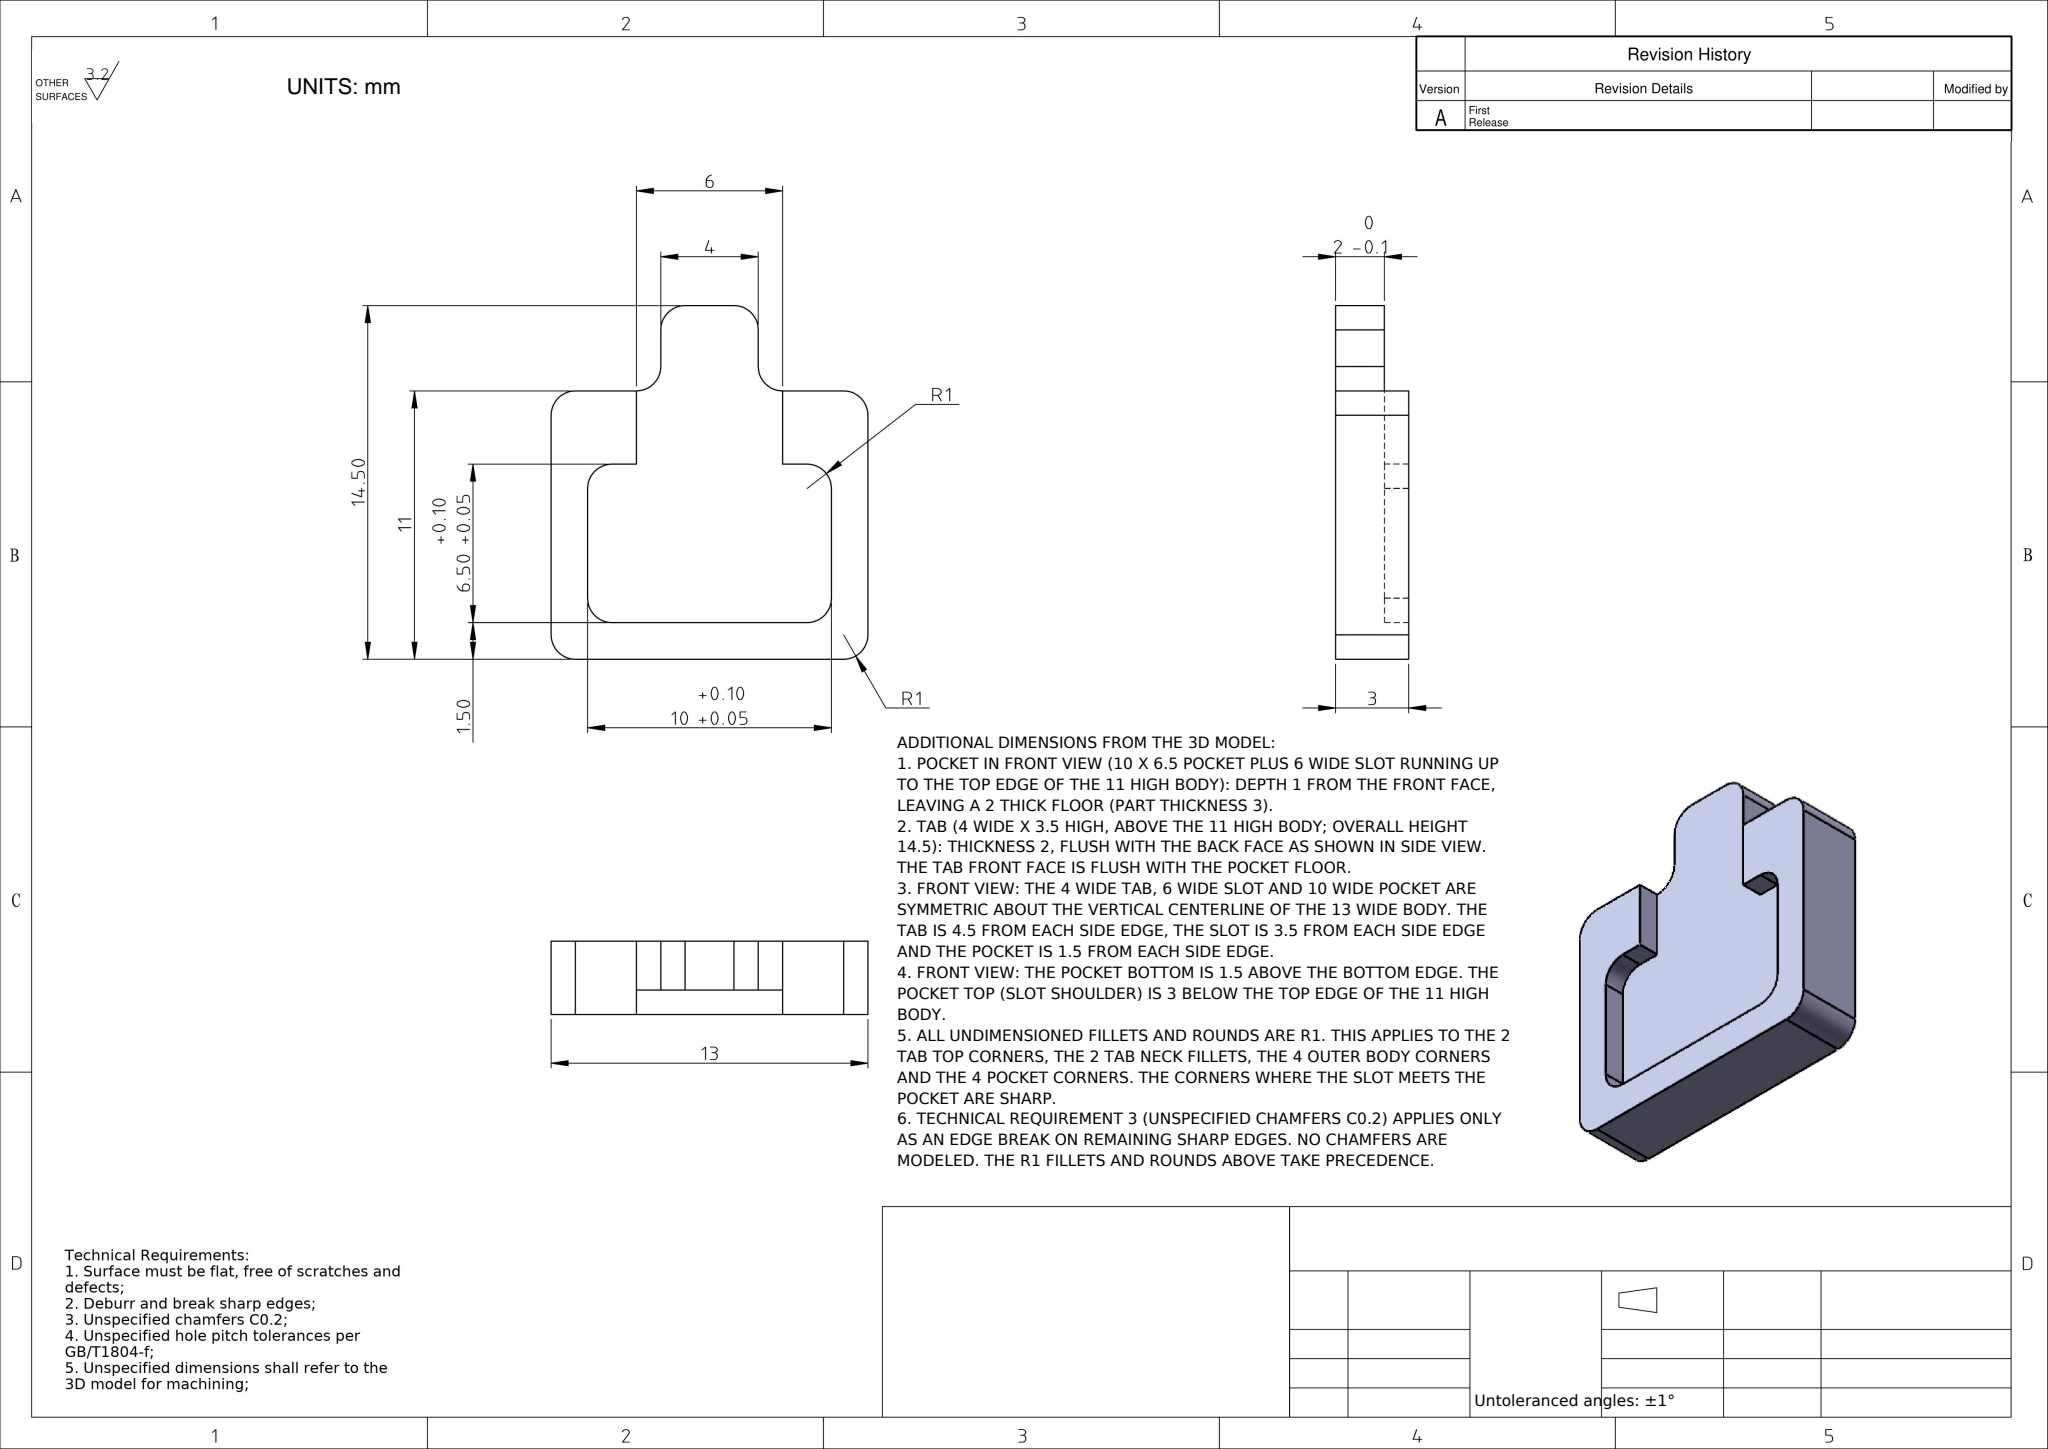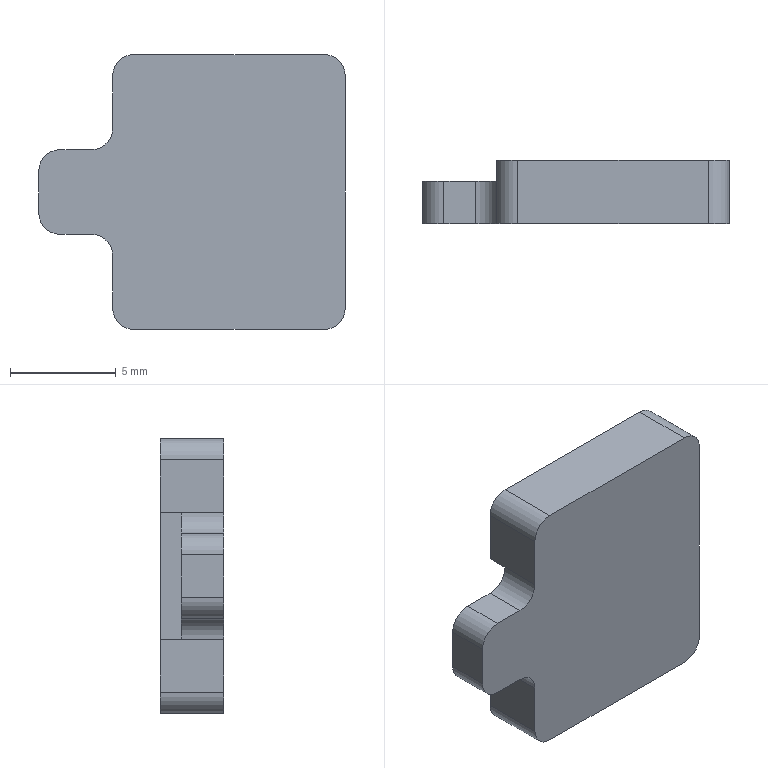Part | NX | mm | 1 solid | 30 faces | box 14.5 x 3 x 13 mm | volume 372 mm3 | plane 18 | cylinder 12 | commonest cylinder face diameters 2 x12
STEP:
#1=COLOUR_RGB('',0.7922,0.8196,0.9333);
#2=FILL_AREA_STYLE_COLOUR('',#1);
#3=FILL_AREA_STYLE('',(#2));
#4=SURFACE_STYLE_FILL_AREA(#3);
#5=SURFACE_SIDE_STYLE('',(#4));
#6=SURFACE_STYLE_USAGE(.BOTH.,#5);
#7=PRESENTATION_STYLE_ASSIGNMENT((#6));
#8=CARTESIAN_POINT('',(-0.75,2.,4.));
#9=VERTEX_POINT('',#8);
#10=CARTESIAN_POINT('',(-0.75,2.,3.));
#11=VERTEX_POINT('',#10);
#12=CARTESIAN_POINT('',(-0.75,2.,3.));
#13=DIRECTION('',(-0.,0.,-1.));
#14=VECTOR('',#13,1000.);
#15=LINE('',#12,#14);
#16=EDGE_CURVE('',#9,#11,#15,.T.);
#17=ORIENTED_EDGE('',*,*,#16,.F.);
#18=CARTESIAN_POINT('',(0.25,2.,5.));
#19=VERTEX_POINT('',#18);
#20=CARTESIAN_POINT('',(0.25,2.,4.));
#21=DIRECTION('',(0.,1.,0.));
#22=DIRECTION('',(0.,0.,-1.));
#23=AXIS2_PLACEMENT_3D('',#20,#21,#22);
#24=CIRCLE('',#23,1.);
#25=EDGE_CURVE('',#9,#19,#24,.T.);
#26=ORIENTED_EDGE('',*,*,#25,.T.);
#27=CARTESIAN_POINT('',(4.75,2.,5.));
#28=VERTEX_POINT('',#27);
#29=CARTESIAN_POINT('',(-0.75,2.,5.));
#30=DIRECTION('',(-1.,0.,0.));
#31=VECTOR('',#30,1000.);
#32=LINE('',#29,#31);
#33=EDGE_CURVE('',#28,#19,#32,.T.);
#34=ORIENTED_EDGE('',*,*,#33,.F.);
#35=CARTESIAN_POINT('',(5.75,2.,4.));
#36=VERTEX_POINT('',#35);
#37=CARTESIAN_POINT('',(4.75,2.,4.));
#38=DIRECTION('',(0.,1.,0.));
#39=DIRECTION('',(0.,0.,-1.));
#40=AXIS2_PLACEMENT_3D('',#37,#38,#39);
#41=CIRCLE('',#40,1.);
#42=EDGE_CURVE('',#28,#36,#41,.T.);
#43=ORIENTED_EDGE('',*,*,#42,.T.);
#44=CARTESIAN_POINT('',(5.75,2.,-4.));
#45=VERTEX_POINT('',#44);
#46=CARTESIAN_POINT('',(5.75,2.,-5.));
#47=DIRECTION('',(0.,0.,1.));
#48=VECTOR('',#47,1000.);
#49=LINE('',#46,#48);
#50=EDGE_CURVE('',#45,#36,#49,.T.);
#51=ORIENTED_EDGE('',*,*,#50,.F.);
#52=CARTESIAN_POINT('',(4.75,2.,-5.));
#53=VERTEX_POINT('',#52);
#54=CARTESIAN_POINT('',(4.75,2.,-4.));
#55=DIRECTION('',(0.,1.,0.));
#56=DIRECTION('',(0.,0.,-1.));
#57=AXIS2_PLACEMENT_3D('',#54,#55,#56);
#58=CIRCLE('',#57,1.);
#59=EDGE_CURVE('',#45,#53,#58,.T.);
#60=ORIENTED_EDGE('',*,*,#59,.T.);
#61=CARTESIAN_POINT('',(0.25,2.,-5.));
#62=VERTEX_POINT('',#61);
#63=CARTESIAN_POINT('',(-0.75,2.,-5.));
#64=DIRECTION('',(1.,0.,0.));
#65=VECTOR('',#64,1000.);
#66=LINE('',#63,#65);
#67=EDGE_CURVE('',#62,#53,#66,.T.);
#68=ORIENTED_EDGE('',*,*,#67,.F.);
#69=CARTESIAN_POINT('',(-0.75,2.,-4.));
#70=VERTEX_POINT('',#69);
#71=CARTESIAN_POINT('',(0.25,2.,-4.));
#72=DIRECTION('',(0.,1.,0.));
#73=DIRECTION('',(0.,0.,-1.));
#74=AXIS2_PLACEMENT_3D('',#71,#72,#73);
#75=CIRCLE('',#74,1.);
#76=EDGE_CURVE('',#62,#70,#75,.T.);
#77=ORIENTED_EDGE('',*,*,#76,.T.);
#78=CARTESIAN_POINT('',(-0.75,2.,-3.));
#79=VERTEX_POINT('',#78);
#80=CARTESIAN_POINT('',(-0.75,2.,-5.));
#81=DIRECTION('',(-0.,0.,-1.));
#82=VECTOR('',#81,1000.);
#83=LINE('',#80,#82);
#84=EDGE_CURVE('',#79,#70,#83,.T.);
#85=ORIENTED_EDGE('',*,*,#84,.F.);
#86=CARTESIAN_POINT('',(-3.75,2.,-3.));
#87=VERTEX_POINT('',#86);
#88=CARTESIAN_POINT('',(-3.75,2.,-3.));
#89=DIRECTION('',(1.,0.,0.));
#90=VECTOR('',#89,1000.);
#91=LINE('',#88,#90);
#92=EDGE_CURVE('',#87,#79,#91,.T.);
#93=ORIENTED_EDGE('',*,*,#92,.F.);
#94=CARTESIAN_POINT('',(-4.75,2.,-2.));
#95=VERTEX_POINT('',#94);
#96=CARTESIAN_POINT('',(-4.75,2.,-3.));
#97=DIRECTION('',(0.,-1.,0.));
#98=DIRECTION('',(0.,0.,-1.));
#99=AXIS2_PLACEMENT_3D('',#96,#97,#98);
#100=CIRCLE('',#99,1.);
#101=EDGE_CURVE('',#87,#95,#100,.T.);
#102=ORIENTED_EDGE('',*,*,#101,.T.);
#103=CARTESIAN_POINT('',(-6.25,2.,-2.));
#104=VERTEX_POINT('',#103);
#105=CARTESIAN_POINT('',(-7.25,2.,-2.));
#106=DIRECTION('',(1.,0.,0.));
#107=VECTOR('',#106,1000.);
#108=LINE('',#105,#107);
#109=EDGE_CURVE('',#104,#95,#108,.T.);
#110=ORIENTED_EDGE('',*,*,#109,.F.);
#111=CARTESIAN_POINT('',(-7.25,2.,-1.));
#112=VERTEX_POINT('',#111);
#113=CARTESIAN_POINT('',(-6.25,2.,-1.));
#114=DIRECTION('',(0.,1.,0.));
#115=DIRECTION('',(0.,0.,-1.));
#116=AXIS2_PLACEMENT_3D('',#113,#114,#115);
#117=CIRCLE('',#116,1.);
#118=EDGE_CURVE('',#104,#112,#117,.T.);
#119=ORIENTED_EDGE('',*,*,#118,.T.);
#120=CARTESIAN_POINT('',(-7.25,2.,1.));
#121=VERTEX_POINT('',#120);
#122=CARTESIAN_POINT('',(-7.25,2.,6.5));
#123=DIRECTION('',(0.,0.,1.));
#124=VECTOR('',#123,1000.);
#125=LINE('',#122,#124);
#126=EDGE_CURVE('',#112,#121,#125,.T.);
#127=ORIENTED_EDGE('',*,*,#126,.T.);
#128=CARTESIAN_POINT('',(-6.25,2.,2.));
#129=VERTEX_POINT('',#128);
#130=CARTESIAN_POINT('',(-6.25,2.,1.));
#131=DIRECTION('',(0.,1.,0.));
#132=DIRECTION('',(0.,0.,-1.));
#133=AXIS2_PLACEMENT_3D('',#130,#131,#132);
#134=CIRCLE('',#133,1.);
#135=EDGE_CURVE('',#121,#129,#134,.T.);
#136=ORIENTED_EDGE('',*,*,#135,.T.);
#137=CARTESIAN_POINT('',(-4.75,2.,2.));
#138=VERTEX_POINT('',#137);
#139=CARTESIAN_POINT('',(-7.25,2.,2.));
#140=DIRECTION('',(-1.,0.,0.));
#141=VECTOR('',#140,1000.);
#142=LINE('',#139,#141);
#143=EDGE_CURVE('',#138,#129,#142,.T.);
#144=ORIENTED_EDGE('',*,*,#143,.F.);
#145=CARTESIAN_POINT('',(-3.75,2.,3.));
#146=VERTEX_POINT('',#145);
#147=CARTESIAN_POINT('',(-4.75,2.,3.));
#148=DIRECTION('',(0.,-1.,0.));
#149=DIRECTION('',(0.,0.,-1.));
#150=AXIS2_PLACEMENT_3D('',#147,#148,#149);
#151=CIRCLE('',#150,1.);
#152=EDGE_CURVE('',#138,#146,#151,.T.);
#153=ORIENTED_EDGE('',*,*,#152,.T.);
#154=CARTESIAN_POINT('',(-3.75,2.,3.));
#155=DIRECTION('',(-1.,0.,0.));
#156=VECTOR('',#155,1000.);
#157=LINE('',#154,#156);
#158=EDGE_CURVE('',#11,#146,#157,.T.);
#159=ORIENTED_EDGE('',*,*,#158,.F.);
#160=EDGE_LOOP('',(#17,#26,#34,#43,#51,#60,#68,#77,#85,#93,#102,#110,#119,#127,#136,#144,#153,#159));
#161=FACE_OUTER_BOUND('',#160,.T.);
#162=CARTESIAN_POINT('',(0.,2.,0.));
#163=DIRECTION('',(0.,-1.,0.));
#164=DIRECTION('',(0.,0.,-1.));
#165=AXIS2_PLACEMENT_3D('',#162,#163,#164);
#166=PLANE('',#165);
#167=ADVANCED_FACE('',(#161),#166,.F.);
#168=CARTESIAN_POINT('',(7.25,0.,5.5));
#169=VERTEX_POINT('',#168);
#170=CARTESIAN_POINT('',(7.25,0.,-5.5));
#171=VERTEX_POINT('',#170);
#172=CARTESIAN_POINT('',(7.25,0.,6.5));
#173=DIRECTION('',(0.,0.,-1.));
#174=VECTOR('',#173,1000.);
#175=LINE('',#172,#174);
#176=EDGE_CURVE('',#169,#171,#175,.T.);
#177=ORIENTED_EDGE('',*,*,#176,.T.);
#178=CARTESIAN_POINT('',(7.25,3.,-5.5));
#179=VERTEX_POINT('',#178);
#180=CARTESIAN_POINT('',(7.25,2.,-5.5));
#181=DIRECTION('',(0.,1.,0.));
#182=VECTOR('',#181,1000.);
#183=LINE('',#180,#182);
#184=EDGE_CURVE('',#171,#179,#183,.T.);
#185=ORIENTED_EDGE('',*,*,#184,.T.);
#186=CARTESIAN_POINT('',(7.25,3.,5.5));
#187=VERTEX_POINT('',#186);
#188=CARTESIAN_POINT('',(7.25,3.,5.5));
#189=DIRECTION('',(0.,0.,-1.));
#190=VECTOR('',#189,1000.);
#191=LINE('',#188,#190);
#192=EDGE_CURVE('',#187,#179,#191,.T.);
#193=ORIENTED_EDGE('',*,*,#192,.F.);
#194=CARTESIAN_POINT('',(7.25,2.,5.5));
#195=DIRECTION('',(0.,-1.,0.));
#196=VECTOR('',#195,1000.);
#197=LINE('',#194,#196);
#198=EDGE_CURVE('',#187,#169,#197,.T.);
#199=ORIENTED_EDGE('',*,*,#198,.T.);
#200=EDGE_LOOP('',(#177,#185,#193,#199));
#201=FACE_OUTER_BOUND('',#200,.T.);
#202=CARTESIAN_POINT('',(7.25,2.,6.5));
#203=DIRECTION('',(-1.,0.,0.));
#204=DIRECTION('',(0.,0.,1.));
#205=AXIS2_PLACEMENT_3D('',#202,#203,#204);
#206=PLANE('',#205);
#207=ADVANCED_FACE('',(#201),#206,.F.);
#208=CARTESIAN_POINT('',(-2.75,0.,-6.5));
#209=VERTEX_POINT('',#208);
#210=CARTESIAN_POINT('',(-2.75,3.,-6.5));
#211=VERTEX_POINT('',#210);
#212=CARTESIAN_POINT('',(-2.75,2.,-6.5));
#213=DIRECTION('',(0.,1.,0.));
#214=VECTOR('',#213,1000.);
#215=LINE('',#212,#214);
#216=EDGE_CURVE('',#209,#211,#215,.T.);
#217=ORIENTED_EDGE('',*,*,#216,.T.);
#218=CARTESIAN_POINT('',(6.25,3.,-6.5));
#219=VERTEX_POINT('',#218);
#220=CARTESIAN_POINT('',(6.25,3.,-6.5));
#221=DIRECTION('',(-1.,0.,0.));
#222=VECTOR('',#221,1000.);
#223=LINE('',#220,#222);
#224=EDGE_CURVE('',#219,#211,#223,.T.);
#225=ORIENTED_EDGE('',*,*,#224,.F.);
#226=CARTESIAN_POINT('',(6.25,0.,-6.5));
#227=VERTEX_POINT('',#226);
#228=CARTESIAN_POINT('',(6.25,2.,-6.5));
#229=DIRECTION('',(0.,-1.,0.));
#230=VECTOR('',#229,1000.);
#231=LINE('',#228,#230);
#232=EDGE_CURVE('',#219,#227,#231,.T.);
#233=ORIENTED_EDGE('',*,*,#232,.T.);
#234=CARTESIAN_POINT('',(-7.25,0.,-6.5));
#235=DIRECTION('',(-1.,0.,0.));
#236=VECTOR('',#235,1000.);
#237=LINE('',#234,#236);
#238=EDGE_CURVE('',#227,#209,#237,.T.);
#239=ORIENTED_EDGE('',*,*,#238,.T.);
#240=EDGE_LOOP('',(#217,#225,#233,#239));
#241=FACE_OUTER_BOUND('',#240,.T.);
#242=CARTESIAN_POINT('',(-7.25,2.,-6.5));
#243=DIRECTION('',(0.,0.,1.));
#244=DIRECTION('',(1.,0.,0.));
#245=AXIS2_PLACEMENT_3D('',#242,#243,#244);
#246=PLANE('',#245);
#247=ADVANCED_FACE('',(#241),#246,.F.);
#248=CARTESIAN_POINT('',(-7.25,0.,-1.));
#249=VERTEX_POINT('',#248);
#250=CARTESIAN_POINT('',(-7.25,0.,1.));
#251=VERTEX_POINT('',#250);
#252=CARTESIAN_POINT('',(-7.25,0.,6.5));
#253=DIRECTION('',(0.,0.,1.));
#254=VECTOR('',#253,1000.);
#255=LINE('',#252,#254);
#256=EDGE_CURVE('',#249,#251,#255,.T.);
#257=ORIENTED_EDGE('',*,*,#256,.T.);
#258=CARTESIAN_POINT('',(-7.25,2.,1.));
#259=DIRECTION('',(0.,1.,0.));
#260=VECTOR('',#259,1000.);
#261=LINE('',#258,#260);
#262=EDGE_CURVE('',#251,#121,#261,.T.);
#263=ORIENTED_EDGE('',*,*,#262,.T.);
#264=ORIENTED_EDGE('',*,*,#126,.F.);
#265=CARTESIAN_POINT('',(-7.25,2.,-1.));
#266=DIRECTION('',(0.,-1.,0.));
#267=VECTOR('',#266,1000.);
#268=LINE('',#265,#267);
#269=EDGE_CURVE('',#112,#249,#268,.T.);
#270=ORIENTED_EDGE('',*,*,#269,.T.);
#271=EDGE_LOOP('',(#257,#263,#264,#270));
#272=FACE_OUTER_BOUND('',#271,.T.);
#273=CARTESIAN_POINT('',(-7.25,2.,6.5));
#274=DIRECTION('',(1.,0.,0.));
#275=DIRECTION('',(0.,0.,-1.));
#276=AXIS2_PLACEMENT_3D('',#273,#274,#275);
#277=PLANE('',#276);
#278=ADVANCED_FACE('',(#272),#277,.F.);
#279=CARTESIAN_POINT('',(-2.75,0.,6.5));
#280=VERTEX_POINT('',#279);
#281=CARTESIAN_POINT('',(6.25,0.,6.5));
#282=VERTEX_POINT('',#281);
#283=CARTESIAN_POINT('',(-7.25,0.,6.5));
#284=DIRECTION('',(1.,0.,0.));
#285=VECTOR('',#284,1000.);
#286=LINE('',#283,#285);
#287=EDGE_CURVE('',#280,#282,#286,.T.);
#288=ORIENTED_EDGE('',*,*,#287,.T.);
#289=CARTESIAN_POINT('',(6.25,3.,6.5));
#290=VERTEX_POINT('',#289);
#291=CARTESIAN_POINT('',(6.25,2.,6.5));
#292=DIRECTION('',(0.,1.,0.));
#293=VECTOR('',#292,1000.);
#294=LINE('',#291,#293);
#295=EDGE_CURVE('',#282,#290,#294,.T.);
#296=ORIENTED_EDGE('',*,*,#295,.T.);
#297=CARTESIAN_POINT('',(-2.75,3.,6.5));
#298=VERTEX_POINT('',#297);
#299=CARTESIAN_POINT('',(-2.75,3.,6.5));
#300=DIRECTION('',(1.,0.,0.));
#301=VECTOR('',#300,1000.);
#302=LINE('',#299,#301);
#303=EDGE_CURVE('',#298,#290,#302,.T.);
#304=ORIENTED_EDGE('',*,*,#303,.F.);
#305=CARTESIAN_POINT('',(-2.75,2.,6.5));
#306=DIRECTION('',(0.,-1.,0.));
#307=VECTOR('',#306,1000.);
#308=LINE('',#305,#307);
#309=EDGE_CURVE('',#298,#280,#308,.T.);
#310=ORIENTED_EDGE('',*,*,#309,.T.);
#311=EDGE_LOOP('',(#288,#296,#304,#310));
#312=FACE_OUTER_BOUND('',#311,.T.);
#313=CARTESIAN_POINT('',(-7.25,2.,6.5));
#314=DIRECTION('',(0.,0.,-1.));
#315=DIRECTION('',(-1.,0.,0.));
#316=AXIS2_PLACEMENT_3D('',#313,#314,#315);
#317=PLANE('',#316);
#318=ADVANCED_FACE('',(#312),#317,.F.);
#319=ORIENTED_EDGE('',*,*,#238,.F.);
#320=CARTESIAN_POINT('',(6.25,0.,-5.5));
#321=DIRECTION('',(0.,-1.,0.));
#322=DIRECTION('',(0.,0.,-1.));
#323=AXIS2_PLACEMENT_3D('',#320,#321,#322);
#324=CIRCLE('',#323,1.);
#325=EDGE_CURVE('',#227,#171,#324,.T.);
#326=ORIENTED_EDGE('',*,*,#325,.T.);
#327=ORIENTED_EDGE('',*,*,#176,.F.);
#328=CARTESIAN_POINT('',(6.25,0.,5.5));
#329=DIRECTION('',(0.,-1.,0.));
#330=DIRECTION('',(0.,0.,-1.));
#331=AXIS2_PLACEMENT_3D('',#328,#329,#330);
#332=CIRCLE('',#331,1.);
#333=EDGE_CURVE('',#169,#282,#332,.T.);
#334=ORIENTED_EDGE('',*,*,#333,.T.);
#335=ORIENTED_EDGE('',*,*,#287,.F.);
#336=CARTESIAN_POINT('',(-3.75,0.,5.5));
#337=VERTEX_POINT('',#336);
#338=CARTESIAN_POINT('',(-2.75,0.,5.5));
#339=DIRECTION('',(0.,-1.,0.));
#340=DIRECTION('',(0.,0.,-1.));
#341=AXIS2_PLACEMENT_3D('',#338,#339,#340);
#342=CIRCLE('',#341,1.);
#343=EDGE_CURVE('',#280,#337,#342,.T.);
#344=ORIENTED_EDGE('',*,*,#343,.T.);
#345=CARTESIAN_POINT('',(-3.75,0.,3.));
#346=VERTEX_POINT('',#345);
#347=CARTESIAN_POINT('',(-3.75,0.,6.5));
#348=DIRECTION('',(0.,0.,-1.));
#349=VECTOR('',#348,1000.);
#350=LINE('',#347,#349);
#351=EDGE_CURVE('',#337,#346,#350,.T.);
#352=ORIENTED_EDGE('',*,*,#351,.T.);
#353=CARTESIAN_POINT('',(-4.75,0.,2.));
#354=VERTEX_POINT('',#353);
#355=CARTESIAN_POINT('',(-4.75,0.,3.));
#356=DIRECTION('',(0.,1.,0.));
#357=DIRECTION('',(0.,0.,-1.));
#358=AXIS2_PLACEMENT_3D('',#355,#356,#357);
#359=CIRCLE('',#358,1.);
#360=EDGE_CURVE('',#346,#354,#359,.T.);
#361=ORIENTED_EDGE('',*,*,#360,.T.);
#362=CARTESIAN_POINT('',(-6.25,0.,2.));
#363=VERTEX_POINT('',#362);
#364=CARTESIAN_POINT('',(-7.25,0.,2.));
#365=DIRECTION('',(-1.,0.,0.));
#366=VECTOR('',#365,1000.);
#367=LINE('',#364,#366);
#368=EDGE_CURVE('',#354,#363,#367,.T.);
#369=ORIENTED_EDGE('',*,*,#368,.T.);
#370=CARTESIAN_POINT('',(-6.25,0.,1.));
#371=DIRECTION('',(0.,-1.,0.));
#372=DIRECTION('',(0.,0.,-1.));
#373=AXIS2_PLACEMENT_3D('',#370,#371,#372);
#374=CIRCLE('',#373,1.);
#375=EDGE_CURVE('',#363,#251,#374,.T.);
#376=ORIENTED_EDGE('',*,*,#375,.T.);
#377=ORIENTED_EDGE('',*,*,#256,.F.);
#378=CARTESIAN_POINT('',(-6.25,0.,-2.));
#379=VERTEX_POINT('',#378);
#380=CARTESIAN_POINT('',(-6.25,0.,-1.));
#381=DIRECTION('',(0.,-1.,0.));
#382=DIRECTION('',(0.,0.,-1.));
#383=AXIS2_PLACEMENT_3D('',#380,#381,#382);
#384=CIRCLE('',#383,1.);
#385=EDGE_CURVE('',#249,#379,#384,.T.);
#386=ORIENTED_EDGE('',*,*,#385,.T.);
#387=CARTESIAN_POINT('',(-4.75,0.,-2.));
#388=VERTEX_POINT('',#387);
#389=CARTESIAN_POINT('',(-7.25,0.,-2.));
#390=DIRECTION('',(1.,0.,0.));
#391=VECTOR('',#390,1000.);
#392=LINE('',#389,#391);
#393=EDGE_CURVE('',#379,#388,#392,.T.);
#394=ORIENTED_EDGE('',*,*,#393,.T.);
#395=CARTESIAN_POINT('',(-3.75,0.,-3.));
#396=VERTEX_POINT('',#395);
#397=CARTESIAN_POINT('',(-4.75,0.,-3.));
#398=DIRECTION('',(0.,1.,0.));
#399=DIRECTION('',(0.,0.,-1.));
#400=AXIS2_PLACEMENT_3D('',#397,#398,#399);
#401=CIRCLE('',#400,1.);
#402=EDGE_CURVE('',#388,#396,#401,.T.);
#403=ORIENTED_EDGE('',*,*,#402,.T.);
#404=CARTESIAN_POINT('',(-3.75,0.,-5.5));
#405=VERTEX_POINT('',#404);
#406=CARTESIAN_POINT('',(-3.75,0.,-6.5));
#407=DIRECTION('',(-0.,0.,-1.));
#408=VECTOR('',#407,1000.);
#409=LINE('',#406,#408);
#410=EDGE_CURVE('',#396,#405,#409,.T.);
#411=ORIENTED_EDGE('',*,*,#410,.T.);
#412=CARTESIAN_POINT('',(-2.75,0.,-5.5));
#413=DIRECTION('',(0.,-1.,0.));
#414=DIRECTION('',(0.,0.,-1.));
#415=AXIS2_PLACEMENT_3D('',#412,#413,#414);
#416=CIRCLE('',#415,1.);
#417=EDGE_CURVE('',#405,#209,#416,.T.);
#418=ORIENTED_EDGE('',*,*,#417,.T.);
#419=EDGE_LOOP('',(#319,#326,#327,#334,#335,#344,#352,#361,#369,#376,#377,#386,#394,#403,#411,#418));
#420=FACE_OUTER_BOUND('',#419,.T.);
#421=CARTESIAN_POINT('',(0.,0.,0.));
#422=DIRECTION('',(0.,-1.,0.));
#423=DIRECTION('',(0.,0.,-1.));
#424=AXIS2_PLACEMENT_3D('',#421,#422,#423);
#425=PLANE('',#424);
#426=ADVANCED_FACE('',(#420),#425,.T.);
#427=ORIENTED_EDGE('',*,*,#410,.F.);
#428=CARTESIAN_POINT('',(-3.75,2.,-3.));
#429=DIRECTION('',(0.,1.,0.));
#430=VECTOR('',#429,1000.);
#431=LINE('',#428,#430);
#432=EDGE_CURVE('',#396,#87,#431,.T.);
#433=ORIENTED_EDGE('',*,*,#432,.T.);
#434=CARTESIAN_POINT('',(-3.75,3.,-3.));
#435=VERTEX_POINT('',#434);
#436=CARTESIAN_POINT('',(-3.75,3.,-3.));
#437=DIRECTION('',(0.,-1.,0.));
#438=VECTOR('',#437,1000.);
#439=LINE('',#436,#438);
#440=EDGE_CURVE('',#435,#87,#439,.T.);
#441=ORIENTED_EDGE('',*,*,#440,.F.);
#442=CARTESIAN_POINT('',(-3.75,3.,-5.5));
#443=VERTEX_POINT('',#442);
#444=CARTESIAN_POINT('',(-3.75,3.,-3.));
#445=DIRECTION('',(0.,0.,1.));
#446=VECTOR('',#445,1000.);
#447=LINE('',#444,#446);
#448=EDGE_CURVE('',#443,#435,#447,.T.);
#449=ORIENTED_EDGE('',*,*,#448,.F.);
#450=CARTESIAN_POINT('',(-3.75,0.,-5.5));
#451=DIRECTION('',(0.,-1.,0.));
#452=VECTOR('',#451,1000.);
#453=LINE('',#450,#452);
#454=EDGE_CURVE('',#443,#405,#453,.T.);
#455=ORIENTED_EDGE('',*,*,#454,.T.);
#456=EDGE_LOOP('',(#427,#433,#441,#449,#455));
#457=FACE_OUTER_BOUND('',#456,.T.);
#458=CARTESIAN_POINT('',(-3.75,0.,-6.5));
#459=DIRECTION('',(1.,0.,-0.));
#460=DIRECTION('',(-0.,0.,-1.));
#461=AXIS2_PLACEMENT_3D('',#458,#459,#460);
#462=PLANE('',#461);
#463=ADVANCED_FACE('',(#457),#462,.F.);
#464=ORIENTED_EDGE('',*,*,#393,.F.);
#465=CARTESIAN_POINT('',(-6.25,0.,-2.));
#466=DIRECTION('',(0.,1.,0.));
#467=VECTOR('',#466,1000.);
#468=LINE('',#465,#467);
#469=EDGE_CURVE('',#379,#104,#468,.T.);
#470=ORIENTED_EDGE('',*,*,#469,.T.);
#471=ORIENTED_EDGE('',*,*,#109,.T.);
#472=CARTESIAN_POINT('',(-4.75,0.,-2.));
#473=DIRECTION('',(0.,-1.,0.));
#474=VECTOR('',#473,1000.);
#475=LINE('',#472,#474);
#476=EDGE_CURVE('',#95,#388,#475,.T.);
#477=ORIENTED_EDGE('',*,*,#476,.T.);
#478=EDGE_LOOP('',(#464,#470,#471,#477));
#479=FACE_OUTER_BOUND('',#478,.T.);
#480=CARTESIAN_POINT('',(-7.25,0.,-2.));
#481=DIRECTION('',(0.,0.,1.));
#482=DIRECTION('',(1.,0.,0.));
#483=AXIS2_PLACEMENT_3D('',#480,#481,#482);
#484=PLANE('',#483);
#485=ADVANCED_FACE('',(#479),#484,.F.);
#486=ORIENTED_EDGE('',*,*,#368,.F.);
#487=CARTESIAN_POINT('',(-4.75,2.,2.));
#488=DIRECTION('',(0.,1.,0.));
#489=VECTOR('',#488,1000.);
#490=LINE('',#487,#489);
#491=EDGE_CURVE('',#354,#138,#490,.T.);
#492=ORIENTED_EDGE('',*,*,#491,.T.);
#493=ORIENTED_EDGE('',*,*,#143,.T.);
#494=CARTESIAN_POINT('',(-6.25,0.,2.));
#495=DIRECTION('',(0.,-1.,0.));
#496=VECTOR('',#495,1000.);
#497=LINE('',#494,#496);
#498=EDGE_CURVE('',#129,#363,#497,.T.);
#499=ORIENTED_EDGE('',*,*,#498,.T.);
#500=EDGE_LOOP('',(#486,#492,#493,#499));
#501=FACE_OUTER_BOUND('',#500,.T.);
#502=CARTESIAN_POINT('',(-7.25,0.,2.));
#503=DIRECTION('',(0.,0.,-1.));
#504=DIRECTION('',(-1.,0.,0.));
#505=AXIS2_PLACEMENT_3D('',#502,#503,#504);
#506=PLANE('',#505);
#507=ADVANCED_FACE('',(#501),#506,.F.);
#508=ORIENTED_EDGE('',*,*,#351,.F.);
#509=CARTESIAN_POINT('',(-3.75,3.,5.5));
#510=VERTEX_POINT('',#509);
#511=CARTESIAN_POINT('',(-3.75,0.,5.5));
#512=DIRECTION('',(0.,1.,0.));
#513=VECTOR('',#512,1000.);
#514=LINE('',#511,#513);
#515=EDGE_CURVE('',#337,#510,#514,.T.);
#516=ORIENTED_EDGE('',*,*,#515,.T.);
#517=CARTESIAN_POINT('',(-3.75,3.,3.));
#518=VERTEX_POINT('',#517);
#519=CARTESIAN_POINT('',(-3.75,3.,5.5));
#520=DIRECTION('',(0.,0.,1.));
#521=VECTOR('',#520,1000.);
#522=LINE('',#519,#521);
#523=EDGE_CURVE('',#518,#510,#522,.T.);
#524=ORIENTED_EDGE('',*,*,#523,.F.);
#525=CARTESIAN_POINT('',(-3.75,3.,3.));
#526=DIRECTION('',(0.,-1.,0.));
#527=VECTOR('',#526,1000.);
#528=LINE('',#525,#527);
#529=EDGE_CURVE('',#518,#146,#528,.T.);
#530=ORIENTED_EDGE('',*,*,#529,.T.);
#531=CARTESIAN_POINT('',(-3.75,0.,3.));
#532=DIRECTION('',(0.,-1.,0.));
#533=VECTOR('',#532,1000.);
#534=LINE('',#531,#533);
#535=EDGE_CURVE('',#146,#346,#534,.T.);
#536=ORIENTED_EDGE('',*,*,#535,.T.);
#537=EDGE_LOOP('',(#508,#516,#524,#530,#536));
#538=FACE_OUTER_BOUND('',#537,.T.);
#539=CARTESIAN_POINT('',(-3.75,0.,6.5));
#540=DIRECTION('',(1.,0.,0.));
#541=DIRECTION('',(0.,0.,-1.));
#542=AXIS2_PLACEMENT_3D('',#539,#540,#541);
#543=PLANE('',#542);
#544=ADVANCED_FACE('',(#538),#543,.F.);
#545=ORIENTED_EDGE('',*,*,#232,.F.);
#546=CARTESIAN_POINT('',(6.25,3.,-5.5));
#547=DIRECTION('',(0.,1.,0.));
#548=DIRECTION('',(0.,0.,1.));
#549=AXIS2_PLACEMENT_3D('',#546,#547,#548);
#550=CIRCLE('',#549,1.);
#551=EDGE_CURVE('',#179,#219,#550,.T.);
#552=ORIENTED_EDGE('',*,*,#551,.F.);
#553=ORIENTED_EDGE('',*,*,#184,.F.);
#554=ORIENTED_EDGE('',*,*,#325,.F.);
#555=EDGE_LOOP('',(#545,#552,#553,#554));
#556=FACE_OUTER_BOUND('',#555,.T.);
#557=CARTESIAN_POINT('',(6.25,2.,-5.5));
#558=DIRECTION('',(0.,-1.,0.));
#559=DIRECTION('',(0.,0.,-1.));
#560=AXIS2_PLACEMENT_3D('',#557,#558,#559);
#561=CYLINDRICAL_SURFACE('',#560,1.);
#562=ADVANCED_FACE('',(#556),#561,.T.);
#563=ORIENTED_EDGE('',*,*,#198,.F.);
#564=CARTESIAN_POINT('',(6.25,3.,5.5));
#565=DIRECTION('',(0.,1.,0.));
#566=DIRECTION('',(0.,0.,1.));
#567=AXIS2_PLACEMENT_3D('',#564,#565,#566);
#568=CIRCLE('',#567,1.);
#569=EDGE_CURVE('',#290,#187,#568,.T.);
#570=ORIENTED_EDGE('',*,*,#569,.F.);
#571=ORIENTED_EDGE('',*,*,#295,.F.);
#572=ORIENTED_EDGE('',*,*,#333,.F.);
#573=EDGE_LOOP('',(#563,#570,#571,#572));
#574=FACE_OUTER_BOUND('',#573,.T.);
#575=CARTESIAN_POINT('',(6.25,2.,5.5));
#576=DIRECTION('',(0.,-1.,0.));
#577=DIRECTION('',(0.,0.,-1.));
#578=AXIS2_PLACEMENT_3D('',#575,#576,#577);
#579=CYLINDRICAL_SURFACE('',#578,1.);
#580=ADVANCED_FACE('',(#574),#579,.T.);
#581=ORIENTED_EDGE('',*,*,#343,.F.);
#582=ORIENTED_EDGE('',*,*,#309,.F.);
#583=CARTESIAN_POINT('',(-2.75,3.,5.5));
#584=DIRECTION('',(0.,1.,0.));
#585=DIRECTION('',(0.,0.,1.));
#586=AXIS2_PLACEMENT_3D('',#583,#584,#585);
#587=CIRCLE('',#586,1.);
#588=EDGE_CURVE('',#510,#298,#587,.T.);
#589=ORIENTED_EDGE('',*,*,#588,.F.);
#590=ORIENTED_EDGE('',*,*,#515,.F.);
#591=EDGE_LOOP('',(#581,#582,#589,#590));
#592=FACE_OUTER_BOUND('',#591,.T.);
#593=CARTESIAN_POINT('',(-2.75,0.,5.5));
#594=DIRECTION('',(0.,1.,0.));
#595=DIRECTION('',(0.,0.,1.));
#596=AXIS2_PLACEMENT_3D('',#593,#594,#595);
#597=CYLINDRICAL_SURFACE('',#596,1.);
#598=ADVANCED_FACE('',(#592),#597,.T.);
#599=ORIENTED_EDGE('',*,*,#360,.F.);
#600=ORIENTED_EDGE('',*,*,#535,.F.);
#601=ORIENTED_EDGE('',*,*,#152,.F.);
#602=ORIENTED_EDGE('',*,*,#491,.F.);
#603=EDGE_LOOP('',(#599,#600,#601,#602));
#604=FACE_OUTER_BOUND('',#603,.T.);
#605=CARTESIAN_POINT('',(-4.75,0.,3.));
#606=DIRECTION('',(0.,-1.,0.));
#607=DIRECTION('',(0.,0.,-1.));
#608=AXIS2_PLACEMENT_3D('',#605,#606,#607);
#609=CYLINDRICAL_SURFACE('',#608,1.);
#610=ADVANCED_FACE('',(#604),#609,.F.);
#611=ORIENTED_EDGE('',*,*,#375,.F.);
#612=ORIENTED_EDGE('',*,*,#498,.F.);
#613=ORIENTED_EDGE('',*,*,#135,.F.);
#614=ORIENTED_EDGE('',*,*,#262,.F.);
#615=EDGE_LOOP('',(#611,#612,#613,#614));
#616=FACE_OUTER_BOUND('',#615,.T.);
#617=CARTESIAN_POINT('',(-6.25,2.,1.));
#618=DIRECTION('',(0.,1.,0.));
#619=DIRECTION('',(0.,0.,1.));
#620=AXIS2_PLACEMENT_3D('',#617,#618,#619);
#621=CYLINDRICAL_SURFACE('',#620,1.);
#622=ADVANCED_FACE('',(#616),#621,.T.);
#623=ORIENTED_EDGE('',*,*,#385,.F.);
#624=ORIENTED_EDGE('',*,*,#269,.F.);
#625=ORIENTED_EDGE('',*,*,#118,.F.);
#626=ORIENTED_EDGE('',*,*,#469,.F.);
#627=EDGE_LOOP('',(#623,#624,#625,#626));
#628=FACE_OUTER_BOUND('',#627,.T.);
#629=CARTESIAN_POINT('',(-6.25,0.,-1.));
#630=DIRECTION('',(0.,1.,0.));
#631=DIRECTION('',(0.,0.,1.));
#632=AXIS2_PLACEMENT_3D('',#629,#630,#631);
#633=CYLINDRICAL_SURFACE('',#632,1.);
#634=ADVANCED_FACE('',(#628),#633,.T.);
#635=ORIENTED_EDGE('',*,*,#402,.F.);
#636=ORIENTED_EDGE('',*,*,#476,.F.);
#637=ORIENTED_EDGE('',*,*,#101,.F.);
#638=ORIENTED_EDGE('',*,*,#432,.F.);
#639=EDGE_LOOP('',(#635,#636,#637,#638));
#640=FACE_OUTER_BOUND('',#639,.T.);
#641=CARTESIAN_POINT('',(-4.75,0.,-3.));
#642=DIRECTION('',(0.,-1.,0.));
#643=DIRECTION('',(0.,0.,-1.));
#644=AXIS2_PLACEMENT_3D('',#641,#642,#643);
#645=CYLINDRICAL_SURFACE('',#644,1.);
#646=ADVANCED_FACE('',(#640),#645,.F.);
#647=ORIENTED_EDGE('',*,*,#417,.F.);
#648=ORIENTED_EDGE('',*,*,#454,.F.);
#649=CARTESIAN_POINT('',(-2.75,3.,-5.5));
#650=DIRECTION('',(0.,1.,0.));
#651=DIRECTION('',(0.,0.,1.));
#652=AXIS2_PLACEMENT_3D('',#649,#650,#651);
#653=CIRCLE('',#652,1.);
#654=EDGE_CURVE('',#211,#443,#653,.T.);
#655=ORIENTED_EDGE('',*,*,#654,.F.);
#656=ORIENTED_EDGE('',*,*,#216,.F.);
#657=EDGE_LOOP('',(#647,#648,#655,#656));
#658=FACE_OUTER_BOUND('',#657,.T.);
#659=CARTESIAN_POINT('',(-2.75,2.,-5.5));
#660=DIRECTION('',(0.,1.,0.));
#661=DIRECTION('',(0.,0.,1.));
#662=AXIS2_PLACEMENT_3D('',#659,#660,#661);
#663=CYLINDRICAL_SURFACE('',#662,1.);
#664=ADVANCED_FACE('',(#658),#663,.T.);
#665=ORIENTED_EDGE('',*,*,#92,.T.);
#666=CARTESIAN_POINT('',(-0.75,3.,-3.));
#667=VERTEX_POINT('',#666);
#668=CARTESIAN_POINT('',(-0.75,3.,-3.));
#669=DIRECTION('',(0.,-1.,0.));
#670=VECTOR('',#669,1000.);
#671=LINE('',#668,#670);
#672=EDGE_CURVE('',#667,#79,#671,.T.);
#673=ORIENTED_EDGE('',*,*,#672,.F.);
#674=CARTESIAN_POINT('',(-3.75,3.,-3.));
#675=DIRECTION('',(1.,0.,0.));
#676=VECTOR('',#675,1000.);
#677=LINE('',#674,#676);
#678=EDGE_CURVE('',#435,#667,#677,.T.);
#679=ORIENTED_EDGE('',*,*,#678,.F.);
#680=ORIENTED_EDGE('',*,*,#440,.T.);
#681=EDGE_LOOP('',(#665,#673,#679,#680));
#682=FACE_OUTER_BOUND('',#681,.T.);
#683=CARTESIAN_POINT('',(-3.75,3.,-3.));
#684=DIRECTION('',(0.,0.,-1.));
#685=DIRECTION('',(-1.,0.,0.));
#686=AXIS2_PLACEMENT_3D('',#683,#684,#685);
#687=PLANE('',#686);
#688=ADVANCED_FACE('',(#682),#687,.F.);
#689=ORIENTED_EDGE('',*,*,#84,.T.);
#690=CARTESIAN_POINT('',(-0.75,3.,-4.));
#691=VERTEX_POINT('',#690);
#692=CARTESIAN_POINT('',(-0.75,3.,-4.));
#693=DIRECTION('',(0.,1.,0.));
#694=VECTOR('',#693,1000.);
#695=LINE('',#692,#694);
#696=EDGE_CURVE('',#70,#691,#695,.T.);
#697=ORIENTED_EDGE('',*,*,#696,.T.);
#698=CARTESIAN_POINT('',(-0.75,3.,-5.));
#699=DIRECTION('',(-0.,0.,-1.));
#700=VECTOR('',#699,1000.);
#701=LINE('',#698,#700);
#702=EDGE_CURVE('',#667,#691,#701,.T.);
#703=ORIENTED_EDGE('',*,*,#702,.F.);
#704=ORIENTED_EDGE('',*,*,#672,.T.);
#705=EDGE_LOOP('',(#689,#697,#703,#704));
#706=FACE_OUTER_BOUND('',#705,.T.);
#707=CARTESIAN_POINT('',(-0.75,3.,-5.));
#708=DIRECTION('',(-1.,0.,0.));
#709=DIRECTION('',(0.,0.,1.));
#710=AXIS2_PLACEMENT_3D('',#707,#708,#709);
#711=PLANE('',#710);
#712=ADVANCED_FACE('',(#706),#711,.F.);
#713=ORIENTED_EDGE('',*,*,#67,.T.);
#714=CARTESIAN_POINT('',(4.75,3.,-5.));
#715=VERTEX_POINT('',#714);
#716=CARTESIAN_POINT('',(4.75,3.,-5.));
#717=DIRECTION('',(0.,1.,0.));
#718=VECTOR('',#717,1000.);
#719=LINE('',#716,#718);
#720=EDGE_CURVE('',#53,#715,#719,.T.);
#721=ORIENTED_EDGE('',*,*,#720,.T.);
#722=CARTESIAN_POINT('',(0.25,3.,-5.));
#723=VERTEX_POINT('',#722);
#724=CARTESIAN_POINT('',(-0.75,3.,-5.));
#725=DIRECTION('',(1.,0.,0.));
#726=VECTOR('',#725,1000.);
#727=LINE('',#724,#726);
#728=EDGE_CURVE('',#723,#715,#727,.T.);
#729=ORIENTED_EDGE('',*,*,#728,.F.);
#730=CARTESIAN_POINT('',(0.25,2.,-5.));
#731=DIRECTION('',(0.,-1.,0.));
#732=VECTOR('',#731,1000.);
#733=LINE('',#730,#732);
#734=EDGE_CURVE('',#723,#62,#733,.T.);
#735=ORIENTED_EDGE('',*,*,#734,.T.);
#736=EDGE_LOOP('',(#713,#721,#729,#735));
#737=FACE_OUTER_BOUND('',#736,.T.);
#738=CARTESIAN_POINT('',(-0.75,3.,-5.));
#739=DIRECTION('',(0.,0.,-1.));
#740=DIRECTION('',(-1.,0.,0.));
#741=AXIS2_PLACEMENT_3D('',#738,#739,#740);
#742=PLANE('',#741);
#743=ADVANCED_FACE('',(#737),#742,.F.);
#744=ORIENTED_EDGE('',*,*,#50,.T.);
#745=CARTESIAN_POINT('',(5.75,3.,4.));
#746=VERTEX_POINT('',#745);
#747=CARTESIAN_POINT('',(5.75,3.,4.));
#748=DIRECTION('',(0.,1.,0.));
#749=VECTOR('',#748,1000.);
#750=LINE('',#747,#749);
#751=EDGE_CURVE('',#36,#746,#750,.T.);
#752=ORIENTED_EDGE('',*,*,#751,.T.);
#753=CARTESIAN_POINT('',(5.75,3.,-4.));
#754=VERTEX_POINT('',#753);
#755=CARTESIAN_POINT('',(5.75,3.,-5.));
#756=DIRECTION('',(0.,0.,1.));
#757=VECTOR('',#756,1000.);
#758=LINE('',#755,#757);
#759=EDGE_CURVE('',#754,#746,#758,.T.);
#760=ORIENTED_EDGE('',*,*,#759,.F.);
#761=CARTESIAN_POINT('',(5.75,2.,-4.));
#762=DIRECTION('',(0.,-1.,0.));
#763=VECTOR('',#762,1000.);
#764=LINE('',#761,#763);
#765=EDGE_CURVE('',#754,#45,#764,.T.);
#766=ORIENTED_EDGE('',*,*,#765,.T.);
#767=EDGE_LOOP('',(#744,#752,#760,#766));
#768=FACE_OUTER_BOUND('',#767,.T.);
#769=CARTESIAN_POINT('',(5.75,3.,-5.));
#770=DIRECTION('',(1.,0.,-0.));
#771=DIRECTION('',(-0.,0.,-1.));
#772=AXIS2_PLACEMENT_3D('',#769,#770,#771);
#773=PLANE('',#772);
#774=ADVANCED_FACE('',(#768),#773,.F.);
#775=ORIENTED_EDGE('',*,*,#33,.T.);
#776=CARTESIAN_POINT('',(0.25,3.,5.));
#777=VERTEX_POINT('',#776);
#778=CARTESIAN_POINT('',(0.25,3.,5.));
#779=DIRECTION('',(0.,1.,0.));
#780=VECTOR('',#779,1000.);
#781=LINE('',#778,#780);
#782=EDGE_CURVE('',#19,#777,#781,.T.);
#783=ORIENTED_EDGE('',*,*,#782,.T.);
#784=CARTESIAN_POINT('',(4.75,3.,5.));
#785=VERTEX_POINT('',#784);
#786=CARTESIAN_POINT('',(-0.75,3.,5.));
#787=DIRECTION('',(-1.,0.,0.));
#788=VECTOR('',#787,1000.);
#789=LINE('',#786,#788);
#790=EDGE_CURVE('',#785,#777,#789,.T.);
#791=ORIENTED_EDGE('',*,*,#790,.F.);
#792=CARTESIAN_POINT('',(4.75,2.,5.));
#793=DIRECTION('',(0.,-1.,0.));
#794=VECTOR('',#793,1000.);
#795=LINE('',#792,#794);
#796=EDGE_CURVE('',#785,#28,#795,.T.);
#797=ORIENTED_EDGE('',*,*,#796,.T.);
#798=EDGE_LOOP('',(#775,#783,#791,#797));
#799=FACE_OUTER_BOUND('',#798,.T.);
#800=CARTESIAN_POINT('',(-0.75,3.,5.));
#801=DIRECTION('',(0.,0.,1.));
#802=DIRECTION('',(1.,0.,-0.));
#803=AXIS2_PLACEMENT_3D('',#800,#801,#802);
#804=PLANE('',#803);
#805=ADVANCED_FACE('',(#799),#804,.F.);
#806=CARTESIAN_POINT('',(-0.75,3.,4.));
#807=VERTEX_POINT('',#806);
#808=CARTESIAN_POINT('',(-0.75,3.,3.));
#809=VERTEX_POINT('',#808);
#810=CARTESIAN_POINT('',(-0.75,3.,3.));
#811=DIRECTION('',(-0.,0.,-1.));
#812=VECTOR('',#811,1000.);
#813=LINE('',#810,#812);
#814=EDGE_CURVE('',#807,#809,#813,.T.);
#815=ORIENTED_EDGE('',*,*,#814,.F.);
#816=CARTESIAN_POINT('',(-0.75,2.,4.));
#817=DIRECTION('',(0.,-1.,0.));
#818=VECTOR('',#817,1000.);
#819=LINE('',#816,#818);
#820=EDGE_CURVE('',#807,#9,#819,.T.);
#821=ORIENTED_EDGE('',*,*,#820,.T.);
#822=ORIENTED_EDGE('',*,*,#16,.T.);
#823=CARTESIAN_POINT('',(-0.75,3.,3.));
#824=DIRECTION('',(0.,-1.,0.));
#825=VECTOR('',#824,1000.);
#826=LINE('',#823,#825);
#827=EDGE_CURVE('',#809,#11,#826,.T.);
#828=ORIENTED_EDGE('',*,*,#827,.F.);
#829=EDGE_LOOP('',(#815,#821,#822,#828));
#830=FACE_OUTER_BOUND('',#829,.T.);
#831=CARTESIAN_POINT('',(-0.75,3.,3.));
#832=DIRECTION('',(-1.,0.,0.));
#833=DIRECTION('',(0.,0.,1.));
#834=AXIS2_PLACEMENT_3D('',#831,#832,#833);
#835=PLANE('',#834);
#836=ADVANCED_FACE('',(#830),#835,.F.);
#837=ORIENTED_EDGE('',*,*,#158,.T.);
#838=ORIENTED_EDGE('',*,*,#529,.F.);
#839=CARTESIAN_POINT('',(-3.75,3.,3.));
#840=DIRECTION('',(-1.,0.,0.));
#841=VECTOR('',#840,1000.);
#842=LINE('',#839,#841);
#843=EDGE_CURVE('',#809,#518,#842,.T.);
#844=ORIENTED_EDGE('',*,*,#843,.F.);
#845=ORIENTED_EDGE('',*,*,#827,.T.);
#846=EDGE_LOOP('',(#837,#838,#844,#845));
#847=FACE_OUTER_BOUND('',#846,.T.);
#848=CARTESIAN_POINT('',(-3.75,3.,3.));
#849=DIRECTION('',(0.,0.,1.));
#850=DIRECTION('',(1.,0.,0.));
#851=AXIS2_PLACEMENT_3D('',#848,#849,#850);
#852=PLANE('',#851);
#853=ADVANCED_FACE('',(#847),#852,.F.);
#854=ORIENTED_EDGE('',*,*,#678,.T.);
#855=ORIENTED_EDGE('',*,*,#702,.T.);
#856=CARTESIAN_POINT('',(0.25,3.,-4.));
#857=DIRECTION('',(0.,-1.,0.));
#858=DIRECTION('',(0.,0.,1.));
#859=AXIS2_PLACEMENT_3D('',#856,#857,#858);
#860=CIRCLE('',#859,1.);
#861=EDGE_CURVE('',#691,#723,#860,.T.);
#862=ORIENTED_EDGE('',*,*,#861,.T.);
#863=ORIENTED_EDGE('',*,*,#728,.T.);
#864=CARTESIAN_POINT('',(4.75,3.,-4.));
#865=DIRECTION('',(0.,-1.,0.));
#866=DIRECTION('',(0.,0.,1.));
#867=AXIS2_PLACEMENT_3D('',#864,#865,#866);
#868=CIRCLE('',#867,1.);
#869=EDGE_CURVE('',#715,#754,#868,.T.);
#870=ORIENTED_EDGE('',*,*,#869,.T.);
#871=ORIENTED_EDGE('',*,*,#759,.T.);
#872=CARTESIAN_POINT('',(4.75,3.,4.));
#873=DIRECTION('',(0.,-1.,0.));
#874=DIRECTION('',(0.,0.,1.));
#875=AXIS2_PLACEMENT_3D('',#872,#873,#874);
#876=CIRCLE('',#875,1.);
#877=EDGE_CURVE('',#746,#785,#876,.T.);
#878=ORIENTED_EDGE('',*,*,#877,.T.);
#879=ORIENTED_EDGE('',*,*,#790,.T.);
#880=CARTESIAN_POINT('',(0.25,3.,4.));
#881=DIRECTION('',(0.,-1.,0.));
#882=DIRECTION('',(0.,0.,1.));
#883=AXIS2_PLACEMENT_3D('',#880,#881,#882);
#884=CIRCLE('',#883,1.);
#885=EDGE_CURVE('',#777,#807,#884,.T.);
#886=ORIENTED_EDGE('',*,*,#885,.T.);
#887=ORIENTED_EDGE('',*,*,#814,.T.);
#888=ORIENTED_EDGE('',*,*,#843,.T.);
#889=ORIENTED_EDGE('',*,*,#523,.T.);
#890=ORIENTED_EDGE('',*,*,#588,.T.);
#891=ORIENTED_EDGE('',*,*,#303,.T.);
#892=ORIENTED_EDGE('',*,*,#569,.T.);
#893=ORIENTED_EDGE('',*,*,#192,.T.);
#894=ORIENTED_EDGE('',*,*,#551,.T.);
#895=ORIENTED_EDGE('',*,*,#224,.T.);
#896=ORIENTED_EDGE('',*,*,#654,.T.);
#897=ORIENTED_EDGE('',*,*,#448,.T.);
#898=EDGE_LOOP('',(#854,#855,#862,#863,#870,#871,#878,#879,#886,#887,#888,#889,#890,#891,#892,#893,#894,#895,#896,#897));
#899=FACE_OUTER_BOUND('',#898,.T.);
#900=CARTESIAN_POINT('',(-2.75,3.,5.5));
#901=DIRECTION('',(0.,1.,0.));
#902=DIRECTION('',(0.,0.,1.));
#903=AXIS2_PLACEMENT_3D('',#900,#901,#902);
#904=PLANE('',#903);
#905=ADVANCED_FACE('',(#899),#904,.T.);
#906=ORIENTED_EDGE('',*,*,#885,.F.);
#907=ORIENTED_EDGE('',*,*,#782,.F.);
#908=ORIENTED_EDGE('',*,*,#25,.F.);
#909=ORIENTED_EDGE('',*,*,#820,.F.);
#910=EDGE_LOOP('',(#906,#907,#908,#909));
#911=FACE_OUTER_BOUND('',#910,.T.);
#912=CARTESIAN_POINT('',(0.25,3.,4.));
#913=DIRECTION('',(0.,1.,0.));
#914=DIRECTION('',(0.,0.,1.));
#915=AXIS2_PLACEMENT_3D('',#912,#913,#914);
#916=CYLINDRICAL_SURFACE('',#915,1.);
#917=ADVANCED_FACE('',(#911),#916,.F.);
#918=ORIENTED_EDGE('',*,*,#877,.F.);
#919=ORIENTED_EDGE('',*,*,#751,.F.);
#920=ORIENTED_EDGE('',*,*,#42,.F.);
#921=ORIENTED_EDGE('',*,*,#796,.F.);
#922=EDGE_LOOP('',(#918,#919,#920,#921));
#923=FACE_OUTER_BOUND('',#922,.T.);
#924=CARTESIAN_POINT('',(4.75,3.,4.));
#925=DIRECTION('',(0.,1.,0.));
#926=DIRECTION('',(0.,0.,1.));
#927=AXIS2_PLACEMENT_3D('',#924,#925,#926);
#928=CYLINDRICAL_SURFACE('',#927,1.);
#929=ADVANCED_FACE('',(#923),#928,.F.);
#930=ORIENTED_EDGE('',*,*,#869,.F.);
#931=ORIENTED_EDGE('',*,*,#720,.F.);
#932=ORIENTED_EDGE('',*,*,#59,.F.);
#933=ORIENTED_EDGE('',*,*,#765,.F.);
#934=EDGE_LOOP('',(#930,#931,#932,#933));
#935=FACE_OUTER_BOUND('',#934,.T.);
#936=CARTESIAN_POINT('',(4.75,3.,-4.));
#937=DIRECTION('',(0.,1.,0.));
#938=DIRECTION('',(0.,0.,1.));
#939=AXIS2_PLACEMENT_3D('',#936,#937,#938);
#940=CYLINDRICAL_SURFACE('',#939,1.);
#941=ADVANCED_FACE('',(#935),#940,.F.);
#942=ORIENTED_EDGE('',*,*,#861,.F.);
#943=ORIENTED_EDGE('',*,*,#696,.F.);
#944=ORIENTED_EDGE('',*,*,#76,.F.);
#945=ORIENTED_EDGE('',*,*,#734,.F.);
#946=EDGE_LOOP('',(#942,#943,#944,#945));
#947=FACE_OUTER_BOUND('',#946,.T.);
#948=CARTESIAN_POINT('',(0.25,3.,-4.));
#949=DIRECTION('',(0.,1.,0.));
#950=DIRECTION('',(0.,0.,1.));
#951=AXIS2_PLACEMENT_3D('',#948,#949,#950);
#952=CYLINDRICAL_SURFACE('',#951,1.);
#953=ADVANCED_FACE('',(#947),#952,.F.);
#954=CLOSED_SHELL('',(#167,#207,#247,#278,#318,#426,#463,#485,#507,#544,#562,#580,#598,#610,#622,#634,#646,#664,#688,#712,#743,#774,#805,#836,#853,#905,#917,#929,#941,#953));
#955=MANIFOLD_SOLID_BREP('',#954);
#956=STYLED_ITEM('',(#7),#955);
#957=(LENGTH_UNIT()NAMED_UNIT(*)SI_UNIT(.MILLI.,.METRE.));
#958=UNCERTAINTY_MEASURE_WITH_UNIT(LENGTH_MEASURE(0.00001),#957,'','');
#959=(NAMED_UNIT(*)PLANE_ANGLE_UNIT()SI_UNIT($,.RADIAN.));
#960=(NAMED_UNIT(*)SI_UNIT($,.STERADIAN.)SOLID_ANGLE_UNIT());
#961=(GEOMETRIC_REPRESENTATION_CONTEXT(3)GLOBAL_UNCERTAINTY_ASSIGNED_CONTEXT((#958))GLOBAL_UNIT_ASSIGNED_CONTEXT((#957,#959,#960))REPRESENTATION_CONTEXT('',''));
#962=MECHANICAL_DESIGN_GEOMETRIC_PRESENTATION_REPRESENTATION('',(#956),#961);
#963=CARTESIAN_POINT('',(0.,0.,0.));
#964=DIRECTION('',(0.,0.,1.));
#965=DIRECTION('',(1.,0.,0.));
#966=AXIS2_PLACEMENT_3D('',#963,#964,#965);
#967=(LENGTH_UNIT()NAMED_UNIT(*)SI_UNIT(.MILLI.,.METRE.));
#968=UNCERTAINTY_MEASURE_WITH_UNIT(LENGTH_MEASURE(0.00001),#967,'','');
#969=(NAMED_UNIT(*)PLANE_ANGLE_UNIT()SI_UNIT($,.RADIAN.));
#970=(NAMED_UNIT(*)SI_UNIT($,.STERADIAN.)SOLID_ANGLE_UNIT());
#971=(GEOMETRIC_REPRESENTATION_CONTEXT(3)GLOBAL_UNCERTAINTY_ASSIGNED_CONTEXT((#968))GLOBAL_UNIT_ASSIGNED_CONTEXT((#967,#969,#970))REPRESENTATION_CONTEXT('',''));
#972=ADVANCED_BREP_SHAPE_REPRESENTATION('',(#955,#966),#971);
#973=PRESENTATION_LAYER_ASSIGNMENT('','',(#956));